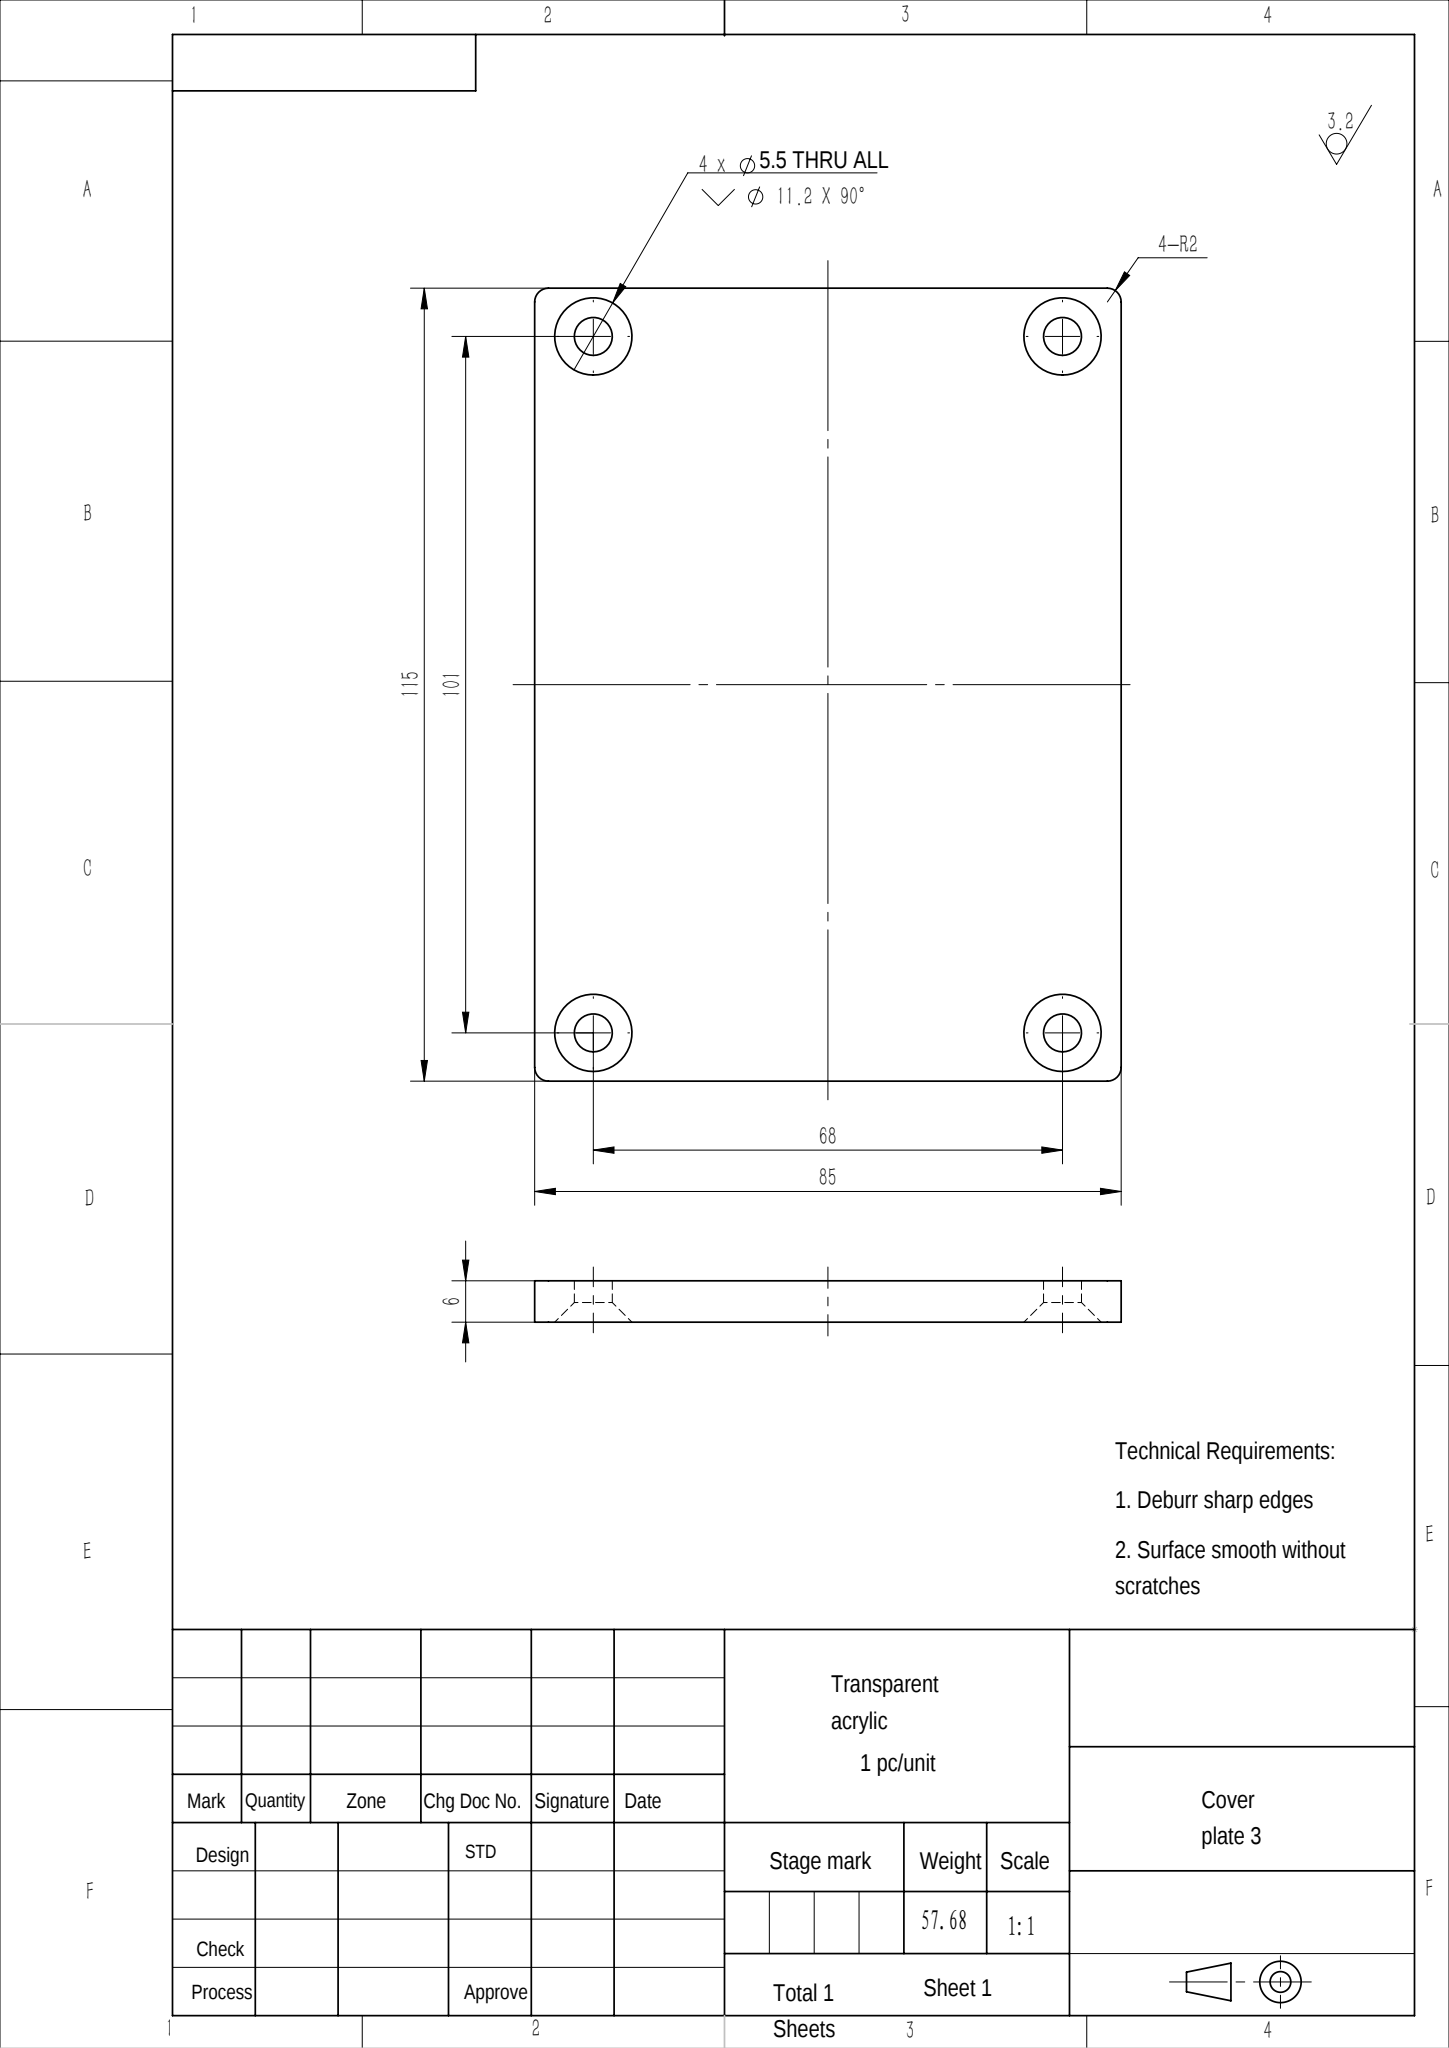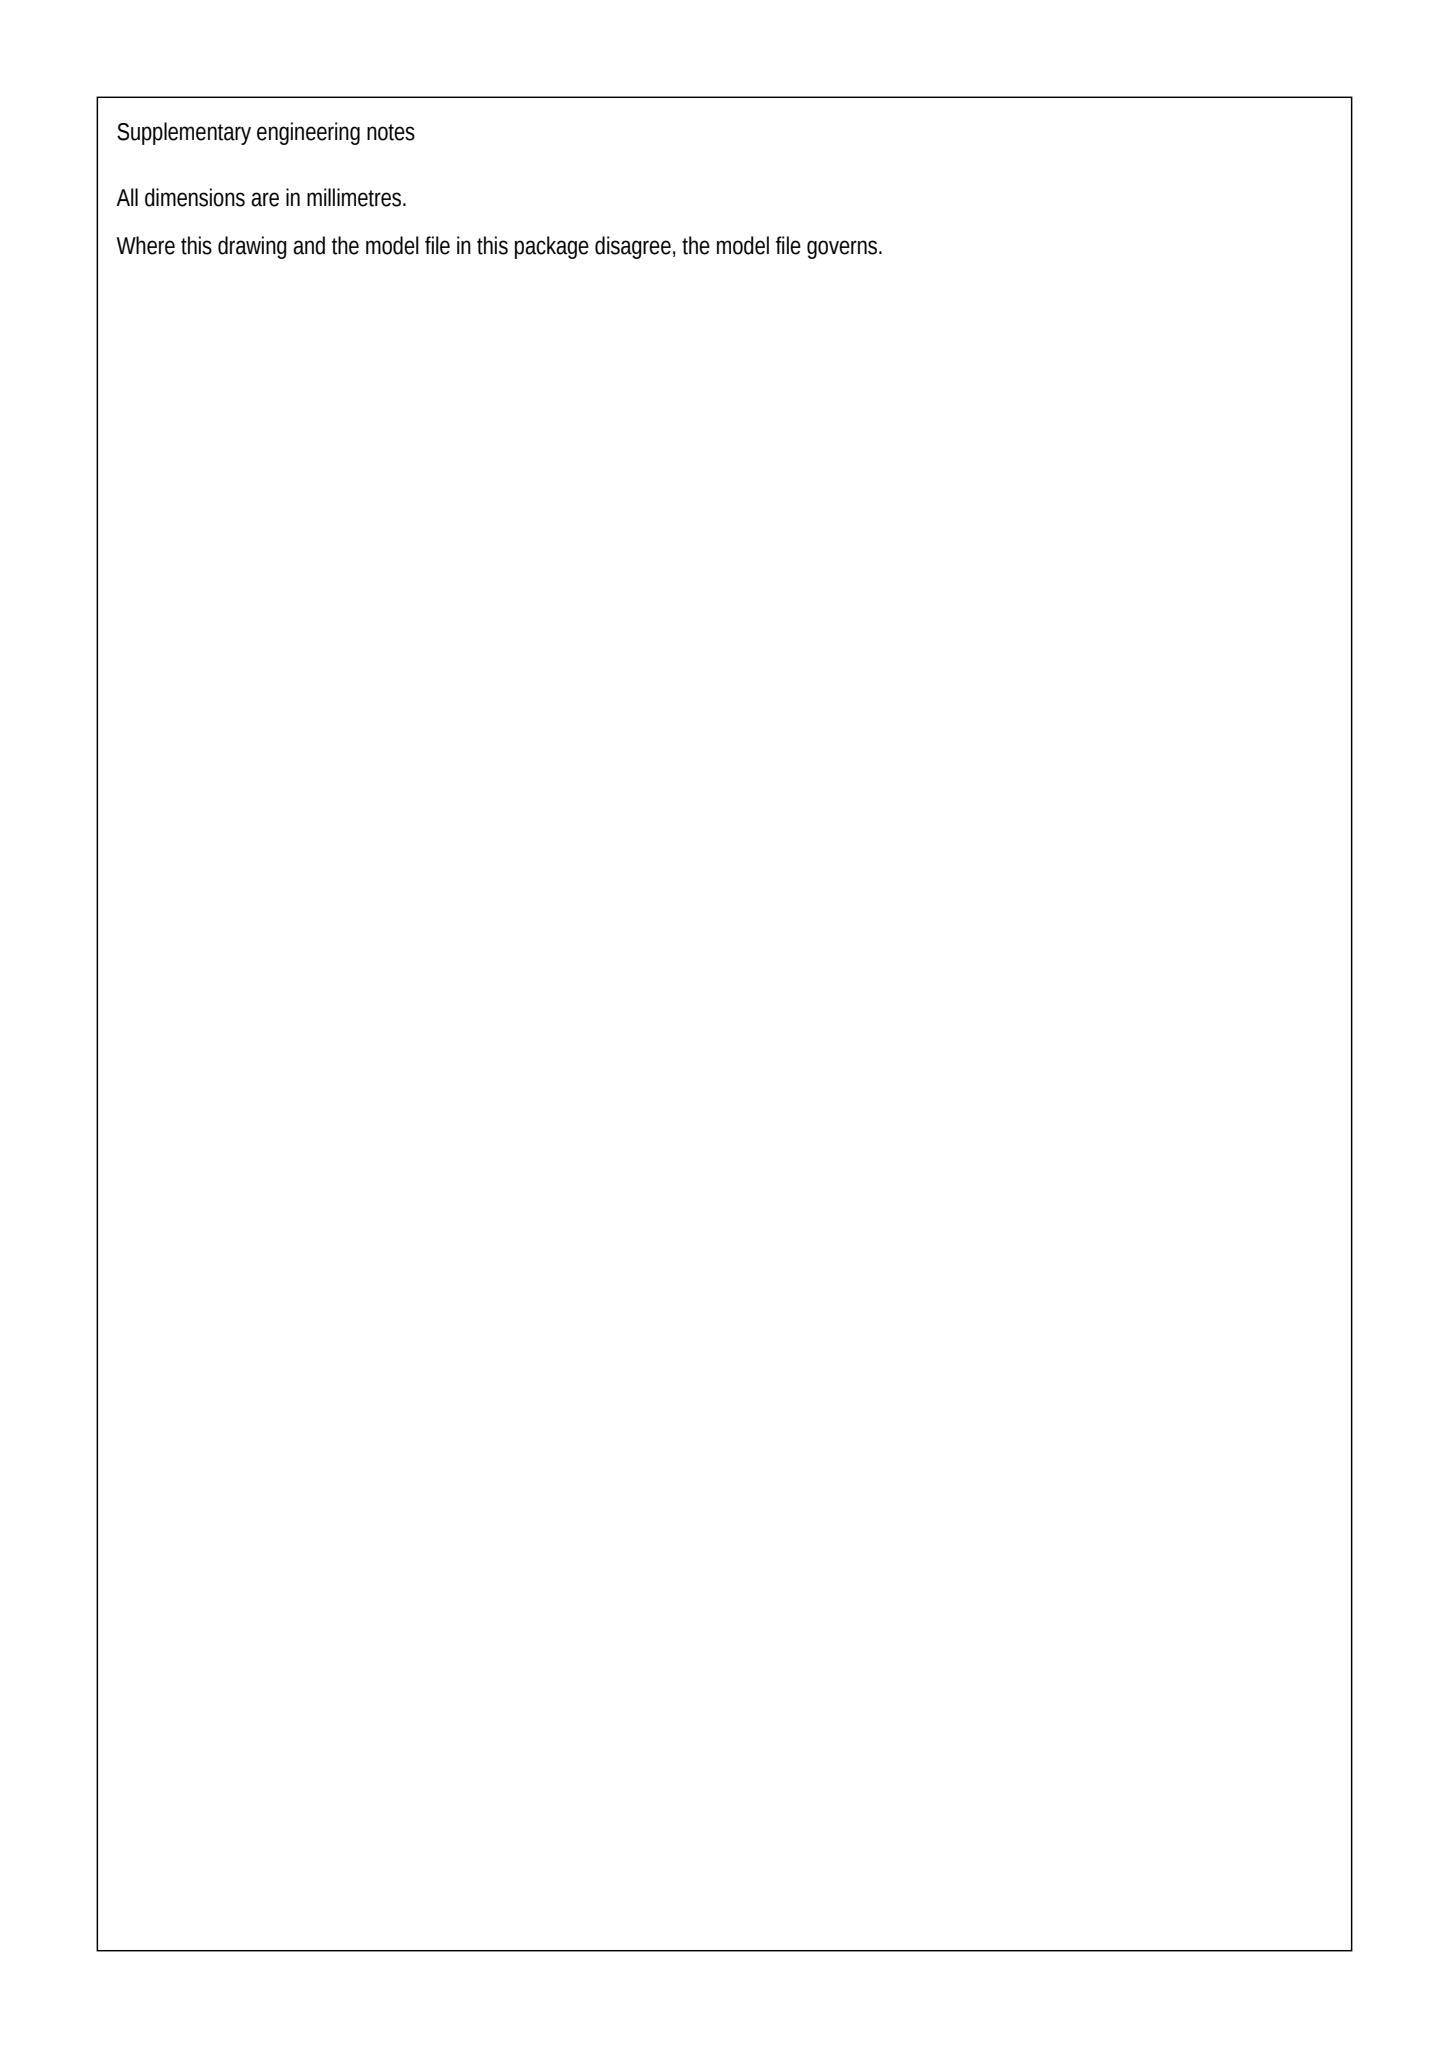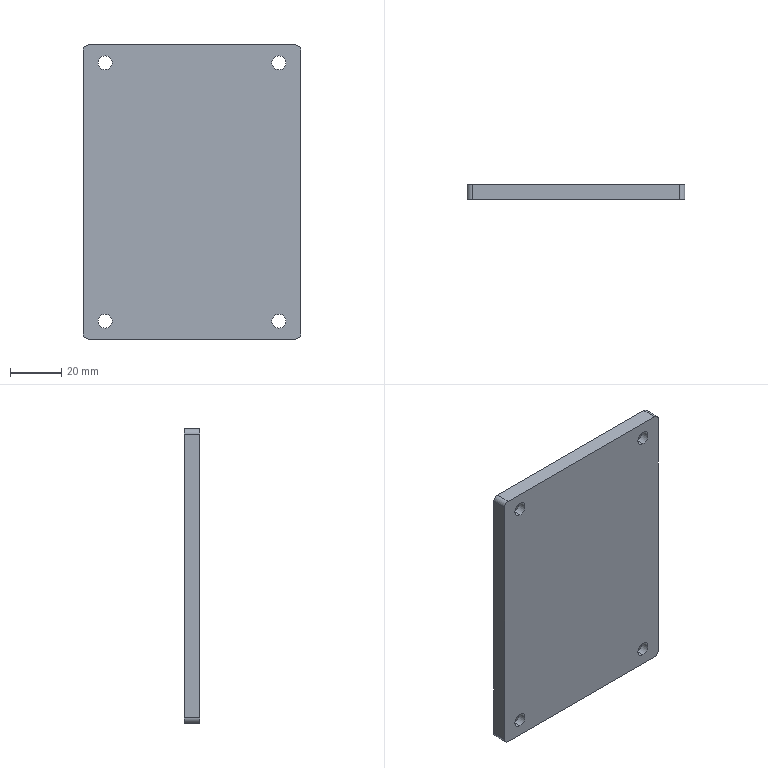Part | SolidWorks | mm | material Transparent acrylic | 1 solid | 26 faces | box 85 x 6 x 115 mm | volume 57682 mm3 | cylinder 12 | cone 8 | plane 6 | commonest cylinder face diameters 5.5 x8 4 x4
build123d program:
from build123d import *

# Parameters (mm, degrees)
SKETCH1_W                                            = 85
SKETCH1_H                                            = 115
BOSS_EXTRUDE1_DEPTH                                  = 6
M5_HEXAGON_SOCKET_COUNTERSUNK_HEAD_SCREW_D           = 5.5
M5_HEXAGON_SOCKET_COUNTERSUNK_HEAD_SCREW_CSINK_D     = 11.2
M5_HEXAGON_SOCKET_COUNTERSUNK_HEAD_SCREW_CSINK_ANGLE = 90
FILLET1_R                                            = 2


with BuildPart() as part:
    # Sketch1 → Boss-Extrude1 (new body)
    with BuildSketch(Plane(origin=(0, 0, 0), x_dir=(1, 0, 0), z_dir=(0, 1, 0))):
        Rectangle(SKETCH1_W, SKETCH1_H)
    extrude(amount=BOSS_EXTRUDE1_DEPTH)

    # M5 Hexagon Socket Countersunk Head Screw (through all)
    with Locations(Plane(origin=(0, 6, 0), x_dir=(1, 0, 0), z_dir=(0, 1, 0))):
        with Locations((-34, 50.5), (-34, -50.5), (34, -50.5), (34, 50.5)):
            CounterSinkHole(M5_HEXAGON_SOCKET_COUNTERSUNK_HEAD_SCREW_D / 2, M5_HEXAGON_SOCKET_COUNTERSUNK_HEAD_SCREW_CSINK_D / 2, counter_sink_angle=M5_HEXAGON_SOCKET_COUNTERSUNK_HEAD_SCREW_CSINK_ANGLE)

    # Fillet1
    fillet1_edges = [part.edges().sort_by_distance(p)[0] for p in [
        (42.5, 3, 57.5),
        (-42.5, 3, 57.5),
        (-42.5, 3, -57.5),
        (42.5, 3, -57.5),
    ]]
    fillet(fillet1_edges, radius=FILLET1_R)


solid = part.part
STEP:
#1=CARTESIAN_POINT('',(-34.,3.15,-53.25));
#2=VERTEX_POINT('',#1);
#3=CARTESIAN_POINT('',(-34.,3.15,-47.75));
#4=VERTEX_POINT('',#3);
#5=CARTESIAN_POINT('',(-34.,3.15,-50.5));
#6=DIRECTION('',(0.,1.,0.));
#7=DIRECTION('',(0.,0.,1.));
#8=AXIS2_PLACEMENT_3D('',#5,#6,#7);
#9=CIRCLE('',#8,2.75);
#10=EDGE_CURVE('',#2,#4,#9,.T.);
#11=ORIENTED_EDGE('',*,*,#10,.F.);
#12=CARTESIAN_POINT('',(-34.,6.,-56.1));
#13=VERTEX_POINT('',#12);
#14=CARTESIAN_POINT('',(-34.,6.,-56.1));
#15=DIRECTION('',(0.,0.7071,-0.7071));
#16=VECTOR('',#15,1000.);
#17=LINE('',#14,#16);
#18=EDGE_CURVE('',#2,#13,#17,.T.);
#19=ORIENTED_EDGE('',*,*,#18,.T.);
#20=CARTESIAN_POINT('',(-34.,6.,-44.9));
#21=VERTEX_POINT('',#20);
#22=CARTESIAN_POINT('',(-34.,6.,-50.5));
#23=DIRECTION('',(0.,1.,0.));
#24=DIRECTION('',(0.,0.,1.));
#25=AXIS2_PLACEMENT_3D('',#22,#23,#24);
#26=CIRCLE('',#25,5.6);
#27=EDGE_CURVE('',#13,#21,#26,.T.);
#28=ORIENTED_EDGE('',*,*,#27,.T.);
#29=CARTESIAN_POINT('',(-34.,6.,-44.9));
#30=DIRECTION('',(0.,0.7071,0.7071));
#31=VECTOR('',#30,1000.);
#32=LINE('',#29,#31);
#33=EDGE_CURVE('',#4,#21,#32,.T.);
#34=ORIENTED_EDGE('',*,*,#33,.F.);
#35=EDGE_LOOP('',(#11,#19,#28,#34));
#36=FACE_OUTER_BOUND('',#35,.T.);
#37=CARTESIAN_POINT('',(-34.,6.,-50.5));
#38=DIRECTION('',(0.,1.,0.));
#39=DIRECTION('',(0.,0.,1.));
#40=AXIS2_PLACEMENT_3D('',#37,#38,#39);
#41=CONICAL_SURFACE('',#40,5.6,0.7854);
#42=ADVANCED_FACE('',(#36),#41,.F.);
#43=CARTESIAN_POINT('',(-34.,-0.,-53.25));
#44=VERTEX_POINT('',#43);
#45=CARTESIAN_POINT('',(-34.,-0.,-47.75));
#46=VERTEX_POINT('',#45);
#47=CARTESIAN_POINT('',(-34.,-0.,-50.5));
#48=DIRECTION('',(0.,1.,0.));
#49=DIRECTION('',(0.,0.,1.));
#50=AXIS2_PLACEMENT_3D('',#47,#48,#49);
#51=CIRCLE('',#50,2.75);
#52=EDGE_CURVE('',#44,#46,#51,.T.);
#53=ORIENTED_EDGE('',*,*,#52,.F.);
#54=CARTESIAN_POINT('',(-34.,6.,-53.25));
#55=DIRECTION('',(0.,1.,0.));
#56=VECTOR('',#55,1000.);
#57=LINE('',#54,#56);
#58=EDGE_CURVE('',#44,#2,#57,.T.);
#59=ORIENTED_EDGE('',*,*,#58,.T.);
#60=ORIENTED_EDGE('',*,*,#10,.T.);
#61=CARTESIAN_POINT('',(-34.,6.,-47.75));
#62=DIRECTION('',(0.,1.,0.));
#63=VECTOR('',#62,1000.);
#64=LINE('',#61,#63);
#65=EDGE_CURVE('',#46,#4,#64,.T.);
#66=ORIENTED_EDGE('',*,*,#65,.F.);
#67=EDGE_LOOP('',(#53,#59,#60,#66));
#68=FACE_OUTER_BOUND('',#67,.T.);
#69=CARTESIAN_POINT('',(-34.,6.,-50.5));
#70=DIRECTION('',(0.,1.,0.));
#71=DIRECTION('',(0.,0.,1.));
#72=AXIS2_PLACEMENT_3D('',#69,#70,#71);
#73=CYLINDRICAL_SURFACE('',#72,2.75);
#74=ADVANCED_FACE('',(#68),#73,.F.);
#75=CARTESIAN_POINT('',(-34.,3.15,47.75));
#76=VERTEX_POINT('',#75);
#77=CARTESIAN_POINT('',(-34.,3.15,53.25));
#78=VERTEX_POINT('',#77);
#79=CARTESIAN_POINT('',(-34.,3.15,50.5));
#80=DIRECTION('',(0.,1.,0.));
#81=DIRECTION('',(0.,0.,1.));
#82=AXIS2_PLACEMENT_3D('',#79,#80,#81);
#83=CIRCLE('',#82,2.75);
#84=EDGE_CURVE('',#76,#78,#83,.T.);
#85=ORIENTED_EDGE('',*,*,#84,.F.);
#86=CARTESIAN_POINT('',(-34.,6.,44.9));
#87=VERTEX_POINT('',#86);
#88=CARTESIAN_POINT('',(-34.,6.,44.9));
#89=DIRECTION('',(0.,0.7071,-0.7071));
#90=VECTOR('',#89,1000.);
#91=LINE('',#88,#90);
#92=EDGE_CURVE('',#76,#87,#91,.T.);
#93=ORIENTED_EDGE('',*,*,#92,.T.);
#94=CARTESIAN_POINT('',(-34.,6.,56.1));
#95=VERTEX_POINT('',#94);
#96=CARTESIAN_POINT('',(-34.,6.,50.5));
#97=DIRECTION('',(0.,1.,0.));
#98=DIRECTION('',(0.,0.,1.));
#99=AXIS2_PLACEMENT_3D('',#96,#97,#98);
#100=CIRCLE('',#99,5.6);
#101=EDGE_CURVE('',#87,#95,#100,.T.);
#102=ORIENTED_EDGE('',*,*,#101,.T.);
#103=CARTESIAN_POINT('',(-34.,6.,56.1));
#104=DIRECTION('',(0.,0.7071,0.7071));
#105=VECTOR('',#104,1000.);
#106=LINE('',#103,#105);
#107=EDGE_CURVE('',#78,#95,#106,.T.);
#108=ORIENTED_EDGE('',*,*,#107,.F.);
#109=EDGE_LOOP('',(#85,#93,#102,#108));
#110=FACE_OUTER_BOUND('',#109,.T.);
#111=CARTESIAN_POINT('',(-34.,6.,50.5));
#112=DIRECTION('',(0.,1.,0.));
#113=DIRECTION('',(0.,0.,1.));
#114=AXIS2_PLACEMENT_3D('',#111,#112,#113);
#115=CONICAL_SURFACE('',#114,5.6,0.7854);
#116=ADVANCED_FACE('',(#110),#115,.F.);
#117=CARTESIAN_POINT('',(-34.,-0.,47.75));
#118=VERTEX_POINT('',#117);
#119=CARTESIAN_POINT('',(-34.,-0.,53.25));
#120=VERTEX_POINT('',#119);
#121=CARTESIAN_POINT('',(-34.,-0.,50.5));
#122=DIRECTION('',(0.,1.,0.));
#123=DIRECTION('',(0.,0.,1.));
#124=AXIS2_PLACEMENT_3D('',#121,#122,#123);
#125=CIRCLE('',#124,2.75);
#126=EDGE_CURVE('',#118,#120,#125,.T.);
#127=ORIENTED_EDGE('',*,*,#126,.F.);
#128=CARTESIAN_POINT('',(-34.,6.,47.75));
#129=DIRECTION('',(0.,1.,0.));
#130=VECTOR('',#129,1000.);
#131=LINE('',#128,#130);
#132=EDGE_CURVE('',#118,#76,#131,.T.);
#133=ORIENTED_EDGE('',*,*,#132,.T.);
#134=ORIENTED_EDGE('',*,*,#84,.T.);
#135=CARTESIAN_POINT('',(-34.,6.,53.25));
#136=DIRECTION('',(0.,1.,0.));
#137=VECTOR('',#136,1000.);
#138=LINE('',#135,#137);
#139=EDGE_CURVE('',#120,#78,#138,.T.);
#140=ORIENTED_EDGE('',*,*,#139,.F.);
#141=EDGE_LOOP('',(#127,#133,#134,#140));
#142=FACE_OUTER_BOUND('',#141,.T.);
#143=CARTESIAN_POINT('',(-34.,6.,50.5));
#144=DIRECTION('',(0.,1.,0.));
#145=DIRECTION('',(0.,0.,1.));
#146=AXIS2_PLACEMENT_3D('',#143,#144,#145);
#147=CYLINDRICAL_SURFACE('',#146,2.75);
#148=ADVANCED_FACE('',(#142),#147,.F.);
#149=CARTESIAN_POINT('',(34.,3.15,47.75));
#150=VERTEX_POINT('',#149);
#151=CARTESIAN_POINT('',(34.,3.15,53.25));
#152=VERTEX_POINT('',#151);
#153=CARTESIAN_POINT('',(34.,3.15,50.5));
#154=DIRECTION('',(0.,1.,0.));
#155=DIRECTION('',(0.,0.,1.));
#156=AXIS2_PLACEMENT_3D('',#153,#154,#155);
#157=CIRCLE('',#156,2.75);
#158=EDGE_CURVE('',#150,#152,#157,.T.);
#159=ORIENTED_EDGE('',*,*,#158,.F.);
#160=CARTESIAN_POINT('',(34.,6.,44.9));
#161=VERTEX_POINT('',#160);
#162=CARTESIAN_POINT('',(34.,6.,44.9));
#163=DIRECTION('',(0.,0.7071,-0.7071));
#164=VECTOR('',#163,1000.);
#165=LINE('',#162,#164);
#166=EDGE_CURVE('',#150,#161,#165,.T.);
#167=ORIENTED_EDGE('',*,*,#166,.T.);
#168=CARTESIAN_POINT('',(34.,6.,56.1));
#169=VERTEX_POINT('',#168);
#170=CARTESIAN_POINT('',(34.,6.,50.5));
#171=DIRECTION('',(0.,1.,0.));
#172=DIRECTION('',(0.,0.,1.));
#173=AXIS2_PLACEMENT_3D('',#170,#171,#172);
#174=CIRCLE('',#173,5.6);
#175=EDGE_CURVE('',#161,#169,#174,.T.);
#176=ORIENTED_EDGE('',*,*,#175,.T.);
#177=CARTESIAN_POINT('',(34.,6.,56.1));
#178=DIRECTION('',(0.,0.7071,0.7071));
#179=VECTOR('',#178,1000.);
#180=LINE('',#177,#179);
#181=EDGE_CURVE('',#152,#169,#180,.T.);
#182=ORIENTED_EDGE('',*,*,#181,.F.);
#183=EDGE_LOOP('',(#159,#167,#176,#182));
#184=FACE_OUTER_BOUND('',#183,.T.);
#185=CARTESIAN_POINT('',(34.,6.,50.5));
#186=DIRECTION('',(0.,1.,0.));
#187=DIRECTION('',(0.,0.,1.));
#188=AXIS2_PLACEMENT_3D('',#185,#186,#187);
#189=CONICAL_SURFACE('',#188,5.6,0.7854);
#190=ADVANCED_FACE('',(#184),#189,.F.);
#191=CARTESIAN_POINT('',(34.,-0.,47.75));
#192=VERTEX_POINT('',#191);
#193=CARTESIAN_POINT('',(34.,-0.,53.25));
#194=VERTEX_POINT('',#193);
#195=CARTESIAN_POINT('',(34.,-0.,50.5));
#196=DIRECTION('',(0.,1.,0.));
#197=DIRECTION('',(0.,0.,1.));
#198=AXIS2_PLACEMENT_3D('',#195,#196,#197);
#199=CIRCLE('',#198,2.75);
#200=EDGE_CURVE('',#192,#194,#199,.T.);
#201=ORIENTED_EDGE('',*,*,#200,.F.);
#202=CARTESIAN_POINT('',(34.,6.,47.75));
#203=DIRECTION('',(0.,1.,0.));
#204=VECTOR('',#203,1000.);
#205=LINE('',#202,#204);
#206=EDGE_CURVE('',#192,#150,#205,.T.);
#207=ORIENTED_EDGE('',*,*,#206,.T.);
#208=ORIENTED_EDGE('',*,*,#158,.T.);
#209=CARTESIAN_POINT('',(34.,6.,53.25));
#210=DIRECTION('',(0.,1.,0.));
#211=VECTOR('',#210,1000.);
#212=LINE('',#209,#211);
#213=EDGE_CURVE('',#194,#152,#212,.T.);
#214=ORIENTED_EDGE('',*,*,#213,.F.);
#215=EDGE_LOOP('',(#201,#207,#208,#214));
#216=FACE_OUTER_BOUND('',#215,.T.);
#217=CARTESIAN_POINT('',(34.,6.,50.5));
#218=DIRECTION('',(0.,1.,0.));
#219=DIRECTION('',(0.,0.,1.));
#220=AXIS2_PLACEMENT_3D('',#217,#218,#219);
#221=CYLINDRICAL_SURFACE('',#220,2.75);
#222=ADVANCED_FACE('',(#216),#221,.F.);
#223=CARTESIAN_POINT('',(34.,3.15,-53.25));
#224=VERTEX_POINT('',#223);
#225=CARTESIAN_POINT('',(34.,3.15,-47.75));
#226=VERTEX_POINT('',#225);
#227=CARTESIAN_POINT('',(34.,3.15,-50.5));
#228=DIRECTION('',(0.,1.,0.));
#229=DIRECTION('',(0.,0.,1.));
#230=AXIS2_PLACEMENT_3D('',#227,#228,#229);
#231=CIRCLE('',#230,2.75);
#232=EDGE_CURVE('',#224,#226,#231,.T.);
#233=ORIENTED_EDGE('',*,*,#232,.F.);
#234=CARTESIAN_POINT('',(34.,6.,-56.1));
#235=VERTEX_POINT('',#234);
#236=CARTESIAN_POINT('',(34.,6.,-56.1));
#237=DIRECTION('',(0.,0.7071,-0.7071));
#238=VECTOR('',#237,1000.);
#239=LINE('',#236,#238);
#240=EDGE_CURVE('',#224,#235,#239,.T.);
#241=ORIENTED_EDGE('',*,*,#240,.T.);
#242=CARTESIAN_POINT('',(34.,6.,-44.9));
#243=VERTEX_POINT('',#242);
#244=CARTESIAN_POINT('',(34.,6.,-50.5));
#245=DIRECTION('',(0.,1.,0.));
#246=DIRECTION('',(0.,0.,1.));
#247=AXIS2_PLACEMENT_3D('',#244,#245,#246);
#248=CIRCLE('',#247,5.6);
#249=EDGE_CURVE('',#235,#243,#248,.T.);
#250=ORIENTED_EDGE('',*,*,#249,.T.);
#251=CARTESIAN_POINT('',(34.,6.,-44.9));
#252=DIRECTION('',(0.,0.7071,0.7071));
#253=VECTOR('',#252,1000.);
#254=LINE('',#251,#253);
#255=EDGE_CURVE('',#226,#243,#254,.T.);
#256=ORIENTED_EDGE('',*,*,#255,.F.);
#257=EDGE_LOOP('',(#233,#241,#250,#256));
#258=FACE_OUTER_BOUND('',#257,.T.);
#259=CARTESIAN_POINT('',(34.,6.,-50.5));
#260=DIRECTION('',(0.,1.,0.));
#261=DIRECTION('',(0.,0.,1.));
#262=AXIS2_PLACEMENT_3D('',#259,#260,#261);
#263=CONICAL_SURFACE('',#262,5.6,0.7854);
#264=ADVANCED_FACE('',(#258),#263,.F.);
#265=CARTESIAN_POINT('',(34.,-0.,-53.25));
#266=VERTEX_POINT('',#265);
#267=CARTESIAN_POINT('',(34.,-0.,-47.75));
#268=VERTEX_POINT('',#267);
#269=CARTESIAN_POINT('',(34.,-0.,-50.5));
#270=DIRECTION('',(0.,1.,0.));
#271=DIRECTION('',(0.,0.,1.));
#272=AXIS2_PLACEMENT_3D('',#269,#270,#271);
#273=CIRCLE('',#272,2.75);
#274=EDGE_CURVE('',#266,#268,#273,.T.);
#275=ORIENTED_EDGE('',*,*,#274,.F.);
#276=CARTESIAN_POINT('',(34.,6.,-53.25));
#277=DIRECTION('',(0.,1.,0.));
#278=VECTOR('',#277,1000.);
#279=LINE('',#276,#278);
#280=EDGE_CURVE('',#266,#224,#279,.T.);
#281=ORIENTED_EDGE('',*,*,#280,.T.);
#282=ORIENTED_EDGE('',*,*,#232,.T.);
#283=CARTESIAN_POINT('',(34.,6.,-47.75));
#284=DIRECTION('',(0.,1.,0.));
#285=VECTOR('',#284,1000.);
#286=LINE('',#283,#285);
#287=EDGE_CURVE('',#268,#226,#286,.T.);
#288=ORIENTED_EDGE('',*,*,#287,.F.);
#289=EDGE_LOOP('',(#275,#281,#282,#288));
#290=FACE_OUTER_BOUND('',#289,.T.);
#291=CARTESIAN_POINT('',(34.,6.,-50.5));
#292=DIRECTION('',(0.,1.,0.));
#293=DIRECTION('',(0.,0.,1.));
#294=AXIS2_PLACEMENT_3D('',#291,#292,#293);
#295=CYLINDRICAL_SURFACE('',#294,2.75);
#296=ADVANCED_FACE('',(#290),#295,.F.);
#297=CARTESIAN_POINT('',(42.5,6.,55.5));
#298=VERTEX_POINT('',#297);
#299=CARTESIAN_POINT('',(42.5,6.,-55.5));
#300=VERTEX_POINT('',#299);
#301=CARTESIAN_POINT('',(42.5,6.,-57.5));
#302=DIRECTION('',(-0.,0.,-1.));
#303=VECTOR('',#302,1000.);
#304=LINE('',#301,#303);
#305=EDGE_CURVE('',#298,#300,#304,.T.);
#306=ORIENTED_EDGE('',*,*,#305,.F.);
#307=CARTESIAN_POINT('',(42.5,0.,55.5));
#308=VERTEX_POINT('',#307);
#309=CARTESIAN_POINT('',(42.5,6.,55.5));
#310=DIRECTION('',(0.,-1.,0.));
#311=VECTOR('',#310,1000.);
#312=LINE('',#309,#311);
#313=EDGE_CURVE('',#298,#308,#312,.T.);
#314=ORIENTED_EDGE('',*,*,#313,.T.);
#315=CARTESIAN_POINT('',(42.5,0.,-55.5));
#316=VERTEX_POINT('',#315);
#317=CARTESIAN_POINT('',(42.5,0.,-57.5));
#318=DIRECTION('',(-0.,0.,-1.));
#319=VECTOR('',#318,1000.);
#320=LINE('',#317,#319);
#321=EDGE_CURVE('',#308,#316,#320,.T.);
#322=ORIENTED_EDGE('',*,*,#321,.T.);
#323=CARTESIAN_POINT('',(42.5,6.,-55.5));
#324=DIRECTION('',(0.,1.,0.));
#325=VECTOR('',#324,1000.);
#326=LINE('',#323,#325);
#327=EDGE_CURVE('',#316,#300,#326,.T.);
#328=ORIENTED_EDGE('',*,*,#327,.T.);
#329=EDGE_LOOP('',(#306,#314,#322,#328));
#330=FACE_OUTER_BOUND('',#329,.T.);
#331=CARTESIAN_POINT('',(42.5,6.,-57.5));
#332=DIRECTION('',(-1.,0.,0.));
#333=DIRECTION('',(0.,0.,1.));
#334=AXIS2_PLACEMENT_3D('',#331,#332,#333);
#335=PLANE('',#334);
#336=ADVANCED_FACE('',(#330),#335,.F.);
#337=CARTESIAN_POINT('',(40.5,6.,-57.5));
#338=VERTEX_POINT('',#337);
#339=CARTESIAN_POINT('',(-40.5,6.,-57.5));
#340=VERTEX_POINT('',#339);
#341=CARTESIAN_POINT('',(-42.5,6.,-57.5));
#342=DIRECTION('',(-1.,0.,0.));
#343=VECTOR('',#342,1000.);
#344=LINE('',#341,#343);
#345=EDGE_CURVE('',#338,#340,#344,.T.);
#346=ORIENTED_EDGE('',*,*,#345,.F.);
#347=CARTESIAN_POINT('',(40.5,0.,-57.5));
#348=VERTEX_POINT('',#347);
#349=CARTESIAN_POINT('',(40.5,6.,-57.5));
#350=DIRECTION('',(0.,-1.,0.));
#351=VECTOR('',#350,1000.);
#352=LINE('',#349,#351);
#353=EDGE_CURVE('',#338,#348,#352,.T.);
#354=ORIENTED_EDGE('',*,*,#353,.T.);
#355=CARTESIAN_POINT('',(-40.5,0.,-57.5));
#356=VERTEX_POINT('',#355);
#357=CARTESIAN_POINT('',(-42.5,0.,-57.5));
#358=DIRECTION('',(-1.,0.,0.));
#359=VECTOR('',#358,1000.);
#360=LINE('',#357,#359);
#361=EDGE_CURVE('',#348,#356,#360,.T.);
#362=ORIENTED_EDGE('',*,*,#361,.T.);
#363=CARTESIAN_POINT('',(-40.5,6.,-57.5));
#364=DIRECTION('',(0.,1.,0.));
#365=VECTOR('',#364,1000.);
#366=LINE('',#363,#365);
#367=EDGE_CURVE('',#356,#340,#366,.T.);
#368=ORIENTED_EDGE('',*,*,#367,.T.);
#369=EDGE_LOOP('',(#346,#354,#362,#368));
#370=FACE_OUTER_BOUND('',#369,.T.);
#371=CARTESIAN_POINT('',(-42.5,6.,-57.5));
#372=DIRECTION('',(0.,0.,1.));
#373=DIRECTION('',(1.,0.,0.));
#374=AXIS2_PLACEMENT_3D('',#371,#372,#373);
#375=PLANE('',#374);
#376=ADVANCED_FACE('',(#370),#375,.F.);
#377=CARTESIAN_POINT('',(-42.5,0.,-55.5));
#378=VERTEX_POINT('',#377);
#379=CARTESIAN_POINT('',(-42.5,0.,55.5));
#380=VERTEX_POINT('',#379);
#381=CARTESIAN_POINT('',(-42.5,0.,-57.5));
#382=DIRECTION('',(0.,0.,1.));
#383=VECTOR('',#382,1000.);
#384=LINE('',#381,#383);
#385=EDGE_CURVE('',#378,#380,#384,.T.);
#386=ORIENTED_EDGE('',*,*,#385,.T.);
#387=CARTESIAN_POINT('',(-42.5,6.,55.5));
#388=VERTEX_POINT('',#387);
#389=CARTESIAN_POINT('',(-42.5,6.,55.5));
#390=DIRECTION('',(0.,1.,0.));
#391=VECTOR('',#390,1000.);
#392=LINE('',#389,#391);
#393=EDGE_CURVE('',#380,#388,#392,.T.);
#394=ORIENTED_EDGE('',*,*,#393,.T.);
#395=CARTESIAN_POINT('',(-42.5,6.,-55.5));
#396=VERTEX_POINT('',#395);
#397=CARTESIAN_POINT('',(-42.5,6.,-57.5));
#398=DIRECTION('',(0.,0.,1.));
#399=VECTOR('',#398,1000.);
#400=LINE('',#397,#399);
#401=EDGE_CURVE('',#396,#388,#400,.T.);
#402=ORIENTED_EDGE('',*,*,#401,.F.);
#403=CARTESIAN_POINT('',(-42.5,6.,-55.5));
#404=DIRECTION('',(0.,-1.,0.));
#405=VECTOR('',#404,1000.);
#406=LINE('',#403,#405);
#407=EDGE_CURVE('',#396,#378,#406,.T.);
#408=ORIENTED_EDGE('',*,*,#407,.T.);
#409=EDGE_LOOP('',(#386,#394,#402,#408));
#410=FACE_OUTER_BOUND('',#409,.T.);
#411=CARTESIAN_POINT('',(-42.5,6.,-57.5));
#412=DIRECTION('',(1.,0.,-0.));
#413=DIRECTION('',(-0.,0.,-1.));
#414=AXIS2_PLACEMENT_3D('',#411,#412,#413);
#415=PLANE('',#414);
#416=ADVANCED_FACE('',(#410),#415,.F.);
#417=CARTESIAN_POINT('',(-40.5,0.,57.5));
#418=VERTEX_POINT('',#417);
#419=CARTESIAN_POINT('',(40.5,0.,57.5));
#420=VERTEX_POINT('',#419);
#421=CARTESIAN_POINT('',(-42.5,0.,57.5));
#422=DIRECTION('',(1.,0.,0.));
#423=VECTOR('',#422,1000.);
#424=LINE('',#421,#423);
#425=EDGE_CURVE('',#418,#420,#424,.T.);
#426=ORIENTED_EDGE('',*,*,#425,.T.);
#427=CARTESIAN_POINT('',(40.5,6.,57.5));
#428=VERTEX_POINT('',#427);
#429=CARTESIAN_POINT('',(40.5,6.,57.5));
#430=DIRECTION('',(0.,1.,0.));
#431=VECTOR('',#430,1000.);
#432=LINE('',#429,#431);
#433=EDGE_CURVE('',#420,#428,#432,.T.);
#434=ORIENTED_EDGE('',*,*,#433,.T.);
#435=CARTESIAN_POINT('',(-40.5,6.,57.5));
#436=VERTEX_POINT('',#435);
#437=CARTESIAN_POINT('',(-42.5,6.,57.5));
#438=DIRECTION('',(1.,0.,0.));
#439=VECTOR('',#438,1000.);
#440=LINE('',#437,#439);
#441=EDGE_CURVE('',#436,#428,#440,.T.);
#442=ORIENTED_EDGE('',*,*,#441,.F.);
#443=CARTESIAN_POINT('',(-40.5,6.,57.5));
#444=DIRECTION('',(0.,-1.,0.));
#445=VECTOR('',#444,1000.);
#446=LINE('',#443,#445);
#447=EDGE_CURVE('',#436,#418,#446,.T.);
#448=ORIENTED_EDGE('',*,*,#447,.T.);
#449=EDGE_LOOP('',(#426,#434,#442,#448));
#450=FACE_OUTER_BOUND('',#449,.T.);
#451=CARTESIAN_POINT('',(-42.5,6.,57.5));
#452=DIRECTION('',(0.,0.,-1.));
#453=DIRECTION('',(-1.,0.,0.));
#454=AXIS2_PLACEMENT_3D('',#451,#452,#453);
#455=PLANE('',#454);
#456=ADVANCED_FACE('',(#450),#455,.F.);
#457=CARTESIAN_POINT('',(-34.,6.,-50.5));
#458=DIRECTION('',(0.,1.,0.));
#459=DIRECTION('',(0.,0.,1.));
#460=AXIS2_PLACEMENT_3D('',#457,#458,#459);
#461=CIRCLE('',#460,5.6);
#462=EDGE_CURVE('',#21,#13,#461,.T.);
#463=ORIENTED_EDGE('',*,*,#462,.F.);
#464=ORIENTED_EDGE('',*,*,#27,.F.);
#465=EDGE_LOOP('',(#463,#464));
#466=FACE_BOUND('',#465,.T.);
#467=CARTESIAN_POINT('',(-34.,6.,50.5));
#468=DIRECTION('',(0.,1.,0.));
#469=DIRECTION('',(0.,0.,1.));
#470=AXIS2_PLACEMENT_3D('',#467,#468,#469);
#471=CIRCLE('',#470,5.6);
#472=EDGE_CURVE('',#95,#87,#471,.T.);
#473=ORIENTED_EDGE('',*,*,#472,.F.);
#474=ORIENTED_EDGE('',*,*,#101,.F.);
#475=EDGE_LOOP('',(#473,#474));
#476=FACE_BOUND('',#475,.T.);
#477=CARTESIAN_POINT('',(34.,6.,50.5));
#478=DIRECTION('',(0.,1.,0.));
#479=DIRECTION('',(0.,0.,1.));
#480=AXIS2_PLACEMENT_3D('',#477,#478,#479);
#481=CIRCLE('',#480,5.6);
#482=EDGE_CURVE('',#169,#161,#481,.T.);
#483=ORIENTED_EDGE('',*,*,#482,.F.);
#484=ORIENTED_EDGE('',*,*,#175,.F.);
#485=EDGE_LOOP('',(#483,#484));
#486=FACE_BOUND('',#485,.T.);
#487=CARTESIAN_POINT('',(34.,6.,-50.5));
#488=DIRECTION('',(0.,1.,0.));
#489=DIRECTION('',(0.,0.,1.));
#490=AXIS2_PLACEMENT_3D('',#487,#488,#489);
#491=CIRCLE('',#490,5.6);
#492=EDGE_CURVE('',#243,#235,#491,.T.);
#493=ORIENTED_EDGE('',*,*,#492,.F.);
#494=ORIENTED_EDGE('',*,*,#249,.F.);
#495=EDGE_LOOP('',(#493,#494));
#496=FACE_BOUND('',#495,.T.);
#497=ORIENTED_EDGE('',*,*,#441,.T.);
#498=CARTESIAN_POINT('',(40.5,6.,55.5));
#499=DIRECTION('',(0.,1.,0.));
#500=DIRECTION('',(0.,0.,1.));
#501=AXIS2_PLACEMENT_3D('',#498,#499,#500);
#502=CIRCLE('',#501,2.);
#503=EDGE_CURVE('',#428,#298,#502,.T.);
#504=ORIENTED_EDGE('',*,*,#503,.T.);
#505=ORIENTED_EDGE('',*,*,#305,.T.);
#506=CARTESIAN_POINT('',(40.5,6.,-55.5));
#507=DIRECTION('',(0.,1.,0.));
#508=DIRECTION('',(0.,0.,1.));
#509=AXIS2_PLACEMENT_3D('',#506,#507,#508);
#510=CIRCLE('',#509,2.);
#511=EDGE_CURVE('',#300,#338,#510,.T.);
#512=ORIENTED_EDGE('',*,*,#511,.T.);
#513=ORIENTED_EDGE('',*,*,#345,.T.);
#514=CARTESIAN_POINT('',(-40.5,6.,-55.5));
#515=DIRECTION('',(0.,1.,0.));
#516=DIRECTION('',(0.,0.,1.));
#517=AXIS2_PLACEMENT_3D('',#514,#515,#516);
#518=CIRCLE('',#517,2.);
#519=EDGE_CURVE('',#340,#396,#518,.T.);
#520=ORIENTED_EDGE('',*,*,#519,.T.);
#521=ORIENTED_EDGE('',*,*,#401,.T.);
#522=CARTESIAN_POINT('',(-40.5,6.,55.5));
#523=DIRECTION('',(0.,1.,0.));
#524=DIRECTION('',(0.,0.,1.));
#525=AXIS2_PLACEMENT_3D('',#522,#523,#524);
#526=CIRCLE('',#525,2.);
#527=EDGE_CURVE('',#388,#436,#526,.T.);
#528=ORIENTED_EDGE('',*,*,#527,.T.);
#529=EDGE_LOOP('',(#497,#504,#505,#512,#513,#520,#521,#528));
#530=FACE_OUTER_BOUND('',#529,.T.);
#531=CARTESIAN_POINT('',(0.,6.,0.));
#532=DIRECTION('',(0.,1.,0.));
#533=DIRECTION('',(0.,0.,1.));
#534=AXIS2_PLACEMENT_3D('',#531,#532,#533);
#535=PLANE('',#534);
#536=ADVANCED_FACE('',(#466,#476,#486,#496,#530),#535,.T.);
#537=CARTESIAN_POINT('',(-34.,-0.,-50.5));
#538=DIRECTION('',(0.,1.,0.));
#539=DIRECTION('',(0.,0.,1.));
#540=AXIS2_PLACEMENT_3D('',#537,#538,#539);
#541=CIRCLE('',#540,2.75);
#542=EDGE_CURVE('',#46,#44,#541,.T.);
#543=ORIENTED_EDGE('',*,*,#542,.T.);
#544=ORIENTED_EDGE('',*,*,#52,.T.);
#545=EDGE_LOOP('',(#543,#544));
#546=FACE_BOUND('',#545,.T.);
#547=CARTESIAN_POINT('',(-34.,-0.,50.5));
#548=DIRECTION('',(0.,1.,0.));
#549=DIRECTION('',(0.,0.,1.));
#550=AXIS2_PLACEMENT_3D('',#547,#548,#549);
#551=CIRCLE('',#550,2.75);
#552=EDGE_CURVE('',#120,#118,#551,.T.);
#553=ORIENTED_EDGE('',*,*,#552,.T.);
#554=ORIENTED_EDGE('',*,*,#126,.T.);
#555=EDGE_LOOP('',(#553,#554));
#556=FACE_BOUND('',#555,.T.);
#557=CARTESIAN_POINT('',(34.,-0.,50.5));
#558=DIRECTION('',(0.,1.,0.));
#559=DIRECTION('',(0.,0.,1.));
#560=AXIS2_PLACEMENT_3D('',#557,#558,#559);
#561=CIRCLE('',#560,2.75);
#562=EDGE_CURVE('',#194,#192,#561,.T.);
#563=ORIENTED_EDGE('',*,*,#562,.T.);
#564=ORIENTED_EDGE('',*,*,#200,.T.);
#565=EDGE_LOOP('',(#563,#564));
#566=FACE_BOUND('',#565,.T.);
#567=CARTESIAN_POINT('',(34.,-0.,-50.5));
#568=DIRECTION('',(0.,1.,0.));
#569=DIRECTION('',(0.,0.,1.));
#570=AXIS2_PLACEMENT_3D('',#567,#568,#569);
#571=CIRCLE('',#570,2.75);
#572=EDGE_CURVE('',#268,#266,#571,.T.);
#573=ORIENTED_EDGE('',*,*,#572,.T.);
#574=ORIENTED_EDGE('',*,*,#274,.T.);
#575=EDGE_LOOP('',(#573,#574));
#576=FACE_BOUND('',#575,.T.);
#577=ORIENTED_EDGE('',*,*,#321,.F.);
#578=CARTESIAN_POINT('',(40.5,0.,55.5));
#579=DIRECTION('',(0.,-1.,0.));
#580=DIRECTION('',(0.,0.,1.));
#581=AXIS2_PLACEMENT_3D('',#578,#579,#580);
#582=CIRCLE('',#581,2.);
#583=EDGE_CURVE('',#308,#420,#582,.T.);
#584=ORIENTED_EDGE('',*,*,#583,.T.);
#585=ORIENTED_EDGE('',*,*,#425,.F.);
#586=CARTESIAN_POINT('',(-40.5,0.,55.5));
#587=DIRECTION('',(0.,-1.,0.));
#588=DIRECTION('',(0.,0.,1.));
#589=AXIS2_PLACEMENT_3D('',#586,#587,#588);
#590=CIRCLE('',#589,2.);
#591=EDGE_CURVE('',#418,#380,#590,.T.);
#592=ORIENTED_EDGE('',*,*,#591,.T.);
#593=ORIENTED_EDGE('',*,*,#385,.F.);
#594=CARTESIAN_POINT('',(-40.5,0.,-55.5));
#595=DIRECTION('',(0.,-1.,0.));
#596=DIRECTION('',(0.,0.,1.));
#597=AXIS2_PLACEMENT_3D('',#594,#595,#596);
#598=CIRCLE('',#597,2.);
#599=EDGE_CURVE('',#378,#356,#598,.T.);
#600=ORIENTED_EDGE('',*,*,#599,.T.);
#601=ORIENTED_EDGE('',*,*,#361,.F.);
#602=CARTESIAN_POINT('',(40.5,0.,-55.5));
#603=DIRECTION('',(0.,-1.,0.));
#604=DIRECTION('',(0.,0.,1.));
#605=AXIS2_PLACEMENT_3D('',#602,#603,#604);
#606=CIRCLE('',#605,2.);
#607=EDGE_CURVE('',#348,#316,#606,.T.);
#608=ORIENTED_EDGE('',*,*,#607,.T.);
#609=EDGE_LOOP('',(#577,#584,#585,#592,#593,#600,#601,#608));
#610=FACE_OUTER_BOUND('',#609,.T.);
#611=CARTESIAN_POINT('',(0.,0.,0.));
#612=DIRECTION('',(0.,1.,0.));
#613=DIRECTION('',(0.,0.,1.));
#614=AXIS2_PLACEMENT_3D('',#611,#612,#613);
#615=PLANE('',#614);
#616=ADVANCED_FACE('',(#546,#556,#566,#576,#610),#615,.F.);
#617=ORIENTED_EDGE('',*,*,#280,.F.);
#618=ORIENTED_EDGE('',*,*,#572,.F.);
#619=ORIENTED_EDGE('',*,*,#287,.T.);
#620=CARTESIAN_POINT('',(34.,3.15,-50.5));
#621=DIRECTION('',(0.,1.,0.));
#622=DIRECTION('',(0.,0.,1.));
#623=AXIS2_PLACEMENT_3D('',#620,#621,#622);
#624=CIRCLE('',#623,2.75);
#625=EDGE_CURVE('',#226,#224,#624,.T.);
#626=ORIENTED_EDGE('',*,*,#625,.T.);
#627=EDGE_LOOP('',(#617,#618,#619,#626));
#628=FACE_OUTER_BOUND('',#627,.T.);
#629=CARTESIAN_POINT('',(34.,6.,-50.5));
#630=DIRECTION('',(0.,1.,0.));
#631=DIRECTION('',(0.,0.,1.));
#632=AXIS2_PLACEMENT_3D('',#629,#630,#631);
#633=CYLINDRICAL_SURFACE('',#632,2.75);
#634=ADVANCED_FACE('',(#628),#633,.F.);
#635=ORIENTED_EDGE('',*,*,#240,.F.);
#636=ORIENTED_EDGE('',*,*,#625,.F.);
#637=ORIENTED_EDGE('',*,*,#255,.T.);
#638=ORIENTED_EDGE('',*,*,#492,.T.);
#639=EDGE_LOOP('',(#635,#636,#637,#638));
#640=FACE_OUTER_BOUND('',#639,.T.);
#641=CARTESIAN_POINT('',(34.,6.,-50.5));
#642=DIRECTION('',(0.,1.,0.));
#643=DIRECTION('',(0.,0.,1.));
#644=AXIS2_PLACEMENT_3D('',#641,#642,#643);
#645=CONICAL_SURFACE('',#644,5.6,0.7854);
#646=ADVANCED_FACE('',(#640),#645,.F.);
#647=ORIENTED_EDGE('',*,*,#206,.F.);
#648=ORIENTED_EDGE('',*,*,#562,.F.);
#649=ORIENTED_EDGE('',*,*,#213,.T.);
#650=CARTESIAN_POINT('',(34.,3.15,50.5));
#651=DIRECTION('',(0.,1.,0.));
#652=DIRECTION('',(0.,0.,1.));
#653=AXIS2_PLACEMENT_3D('',#650,#651,#652);
#654=CIRCLE('',#653,2.75);
#655=EDGE_CURVE('',#152,#150,#654,.T.);
#656=ORIENTED_EDGE('',*,*,#655,.T.);
#657=EDGE_LOOP('',(#647,#648,#649,#656));
#658=FACE_OUTER_BOUND('',#657,.T.);
#659=CARTESIAN_POINT('',(34.,6.,50.5));
#660=DIRECTION('',(0.,1.,0.));
#661=DIRECTION('',(0.,0.,1.));
#662=AXIS2_PLACEMENT_3D('',#659,#660,#661);
#663=CYLINDRICAL_SURFACE('',#662,2.75);
#664=ADVANCED_FACE('',(#658),#663,.F.);
#665=ORIENTED_EDGE('',*,*,#166,.F.);
#666=ORIENTED_EDGE('',*,*,#655,.F.);
#667=ORIENTED_EDGE('',*,*,#181,.T.);
#668=ORIENTED_EDGE('',*,*,#482,.T.);
#669=EDGE_LOOP('',(#665,#666,#667,#668));
#670=FACE_OUTER_BOUND('',#669,.T.);
#671=CARTESIAN_POINT('',(34.,6.,50.5));
#672=DIRECTION('',(0.,1.,0.));
#673=DIRECTION('',(0.,0.,1.));
#674=AXIS2_PLACEMENT_3D('',#671,#672,#673);
#675=CONICAL_SURFACE('',#674,5.6,0.7854);
#676=ADVANCED_FACE('',(#670),#675,.F.);
#677=ORIENTED_EDGE('',*,*,#132,.F.);
#678=ORIENTED_EDGE('',*,*,#552,.F.);
#679=ORIENTED_EDGE('',*,*,#139,.T.);
#680=CARTESIAN_POINT('',(-34.,3.15,50.5));
#681=DIRECTION('',(0.,1.,0.));
#682=DIRECTION('',(0.,0.,1.));
#683=AXIS2_PLACEMENT_3D('',#680,#681,#682);
#684=CIRCLE('',#683,2.75);
#685=EDGE_CURVE('',#78,#76,#684,.T.);
#686=ORIENTED_EDGE('',*,*,#685,.T.);
#687=EDGE_LOOP('',(#677,#678,#679,#686));
#688=FACE_OUTER_BOUND('',#687,.T.);
#689=CARTESIAN_POINT('',(-34.,6.,50.5));
#690=DIRECTION('',(0.,1.,0.));
#691=DIRECTION('',(0.,0.,1.));
#692=AXIS2_PLACEMENT_3D('',#689,#690,#691);
#693=CYLINDRICAL_SURFACE('',#692,2.75);
#694=ADVANCED_FACE('',(#688),#693,.F.);
#695=ORIENTED_EDGE('',*,*,#92,.F.);
#696=ORIENTED_EDGE('',*,*,#685,.F.);
#697=ORIENTED_EDGE('',*,*,#107,.T.);
#698=ORIENTED_EDGE('',*,*,#472,.T.);
#699=EDGE_LOOP('',(#695,#696,#697,#698));
#700=FACE_OUTER_BOUND('',#699,.T.);
#701=CARTESIAN_POINT('',(-34.,6.,50.5));
#702=DIRECTION('',(0.,1.,0.));
#703=DIRECTION('',(0.,0.,1.));
#704=AXIS2_PLACEMENT_3D('',#701,#702,#703);
#705=CONICAL_SURFACE('',#704,5.6,0.7854);
#706=ADVANCED_FACE('',(#700),#705,.F.);
#707=ORIENTED_EDGE('',*,*,#58,.F.);
#708=ORIENTED_EDGE('',*,*,#542,.F.);
#709=ORIENTED_EDGE('',*,*,#65,.T.);
#710=CARTESIAN_POINT('',(-34.,3.15,-50.5));
#711=DIRECTION('',(0.,1.,0.));
#712=DIRECTION('',(0.,0.,1.));
#713=AXIS2_PLACEMENT_3D('',#710,#711,#712);
#714=CIRCLE('',#713,2.75);
#715=EDGE_CURVE('',#4,#2,#714,.T.);
#716=ORIENTED_EDGE('',*,*,#715,.T.);
#717=EDGE_LOOP('',(#707,#708,#709,#716));
#718=FACE_OUTER_BOUND('',#717,.T.);
#719=CARTESIAN_POINT('',(-34.,6.,-50.5));
#720=DIRECTION('',(0.,1.,0.));
#721=DIRECTION('',(0.,0.,1.));
#722=AXIS2_PLACEMENT_3D('',#719,#720,#721);
#723=CYLINDRICAL_SURFACE('',#722,2.75);
#724=ADVANCED_FACE('',(#718),#723,.F.);
#725=ORIENTED_EDGE('',*,*,#18,.F.);
#726=ORIENTED_EDGE('',*,*,#715,.F.);
#727=ORIENTED_EDGE('',*,*,#33,.T.);
#728=ORIENTED_EDGE('',*,*,#462,.T.);
#729=EDGE_LOOP('',(#725,#726,#727,#728));
#730=FACE_OUTER_BOUND('',#729,.T.);
#731=CARTESIAN_POINT('',(-34.,6.,-50.5));
#732=DIRECTION('',(0.,1.,0.));
#733=DIRECTION('',(0.,0.,1.));
#734=AXIS2_PLACEMENT_3D('',#731,#732,#733);
#735=CONICAL_SURFACE('',#734,5.6,0.7854);
#736=ADVANCED_FACE('',(#730),#735,.F.);
#737=ORIENTED_EDGE('',*,*,#503,.F.);
#738=ORIENTED_EDGE('',*,*,#433,.F.);
#739=ORIENTED_EDGE('',*,*,#583,.F.);
#740=ORIENTED_EDGE('',*,*,#313,.F.);
#741=EDGE_LOOP('',(#737,#738,#739,#740));
#742=FACE_OUTER_BOUND('',#741,.T.);
#743=CARTESIAN_POINT('',(40.5,6.,55.5));
#744=DIRECTION('',(0.,-1.,0.));
#745=DIRECTION('',(0.,0.,-1.));
#746=AXIS2_PLACEMENT_3D('',#743,#744,#745);
#747=CYLINDRICAL_SURFACE('',#746,2.);
#748=ADVANCED_FACE('',(#742),#747,.T.);
#749=ORIENTED_EDGE('',*,*,#527,.F.);
#750=ORIENTED_EDGE('',*,*,#393,.F.);
#751=ORIENTED_EDGE('',*,*,#591,.F.);
#752=ORIENTED_EDGE('',*,*,#447,.F.);
#753=EDGE_LOOP('',(#749,#750,#751,#752));
#754=FACE_OUTER_BOUND('',#753,.T.);
#755=CARTESIAN_POINT('',(-40.5,6.,55.5));
#756=DIRECTION('',(0.,-1.,0.));
#757=DIRECTION('',(0.,0.,-1.));
#758=AXIS2_PLACEMENT_3D('',#755,#756,#757);
#759=CYLINDRICAL_SURFACE('',#758,2.);
#760=ADVANCED_FACE('',(#754),#759,.T.);
#761=ORIENTED_EDGE('',*,*,#511,.F.);
#762=ORIENTED_EDGE('',*,*,#327,.F.);
#763=ORIENTED_EDGE('',*,*,#607,.F.);
#764=ORIENTED_EDGE('',*,*,#353,.F.);
#765=EDGE_LOOP('',(#761,#762,#763,#764));
#766=FACE_OUTER_BOUND('',#765,.T.);
#767=CARTESIAN_POINT('',(40.5,6.,-55.5));
#768=DIRECTION('',(0.,-1.,0.));
#769=DIRECTION('',(0.,0.,-1.));
#770=AXIS2_PLACEMENT_3D('',#767,#768,#769);
#771=CYLINDRICAL_SURFACE('',#770,2.);
#772=ADVANCED_FACE('',(#766),#771,.T.);
#773=ORIENTED_EDGE('',*,*,#519,.F.);
#774=ORIENTED_EDGE('',*,*,#367,.F.);
#775=ORIENTED_EDGE('',*,*,#599,.F.);
#776=ORIENTED_EDGE('',*,*,#407,.F.);
#777=EDGE_LOOP('',(#773,#774,#775,#776));
#778=FACE_OUTER_BOUND('',#777,.T.);
#779=CARTESIAN_POINT('',(-40.5,6.,-55.5));
#780=DIRECTION('',(0.,-1.,0.));
#781=DIRECTION('',(0.,0.,-1.));
#782=AXIS2_PLACEMENT_3D('',#779,#780,#781);
#783=CYLINDRICAL_SURFACE('',#782,2.);
#784=ADVANCED_FACE('',(#778),#783,.T.);
#785=CLOSED_SHELL('',(#42,#74,#116,#148,#190,#222,#264,#296,#336,#376,#416,#456,#536,#616,#634,#646,#664,#676,#694,#706,#724,#736,#748,#760,#772,#784));
#786=MANIFOLD_SOLID_BREP('',#785);
#787=CARTESIAN_POINT('',(0.,0.,0.));
#788=DIRECTION('',(0.,0.,1.));
#789=DIRECTION('',(1.,0.,0.));
#790=AXIS2_PLACEMENT_3D('',#787,#788,#789);
#791=(LENGTH_UNIT()NAMED_UNIT(*)SI_UNIT(.MILLI.,.METRE.));
#792=UNCERTAINTY_MEASURE_WITH_UNIT(LENGTH_MEASURE(0.00001),#791,'','');
#793=(NAMED_UNIT(*)PLANE_ANGLE_UNIT()SI_UNIT($,.RADIAN.));
#794=(NAMED_UNIT(*)SI_UNIT($,.STERADIAN.)SOLID_ANGLE_UNIT());
#795=(GEOMETRIC_REPRESENTATION_CONTEXT(3)GLOBAL_UNCERTAINTY_ASSIGNED_CONTEXT((#792))GLOBAL_UNIT_ASSIGNED_CONTEXT((#791,#793,#794))REPRESENTATION_CONTEXT('',''));
#796=ADVANCED_BREP_SHAPE_REPRESENTATION('',(#786,#790),#795);